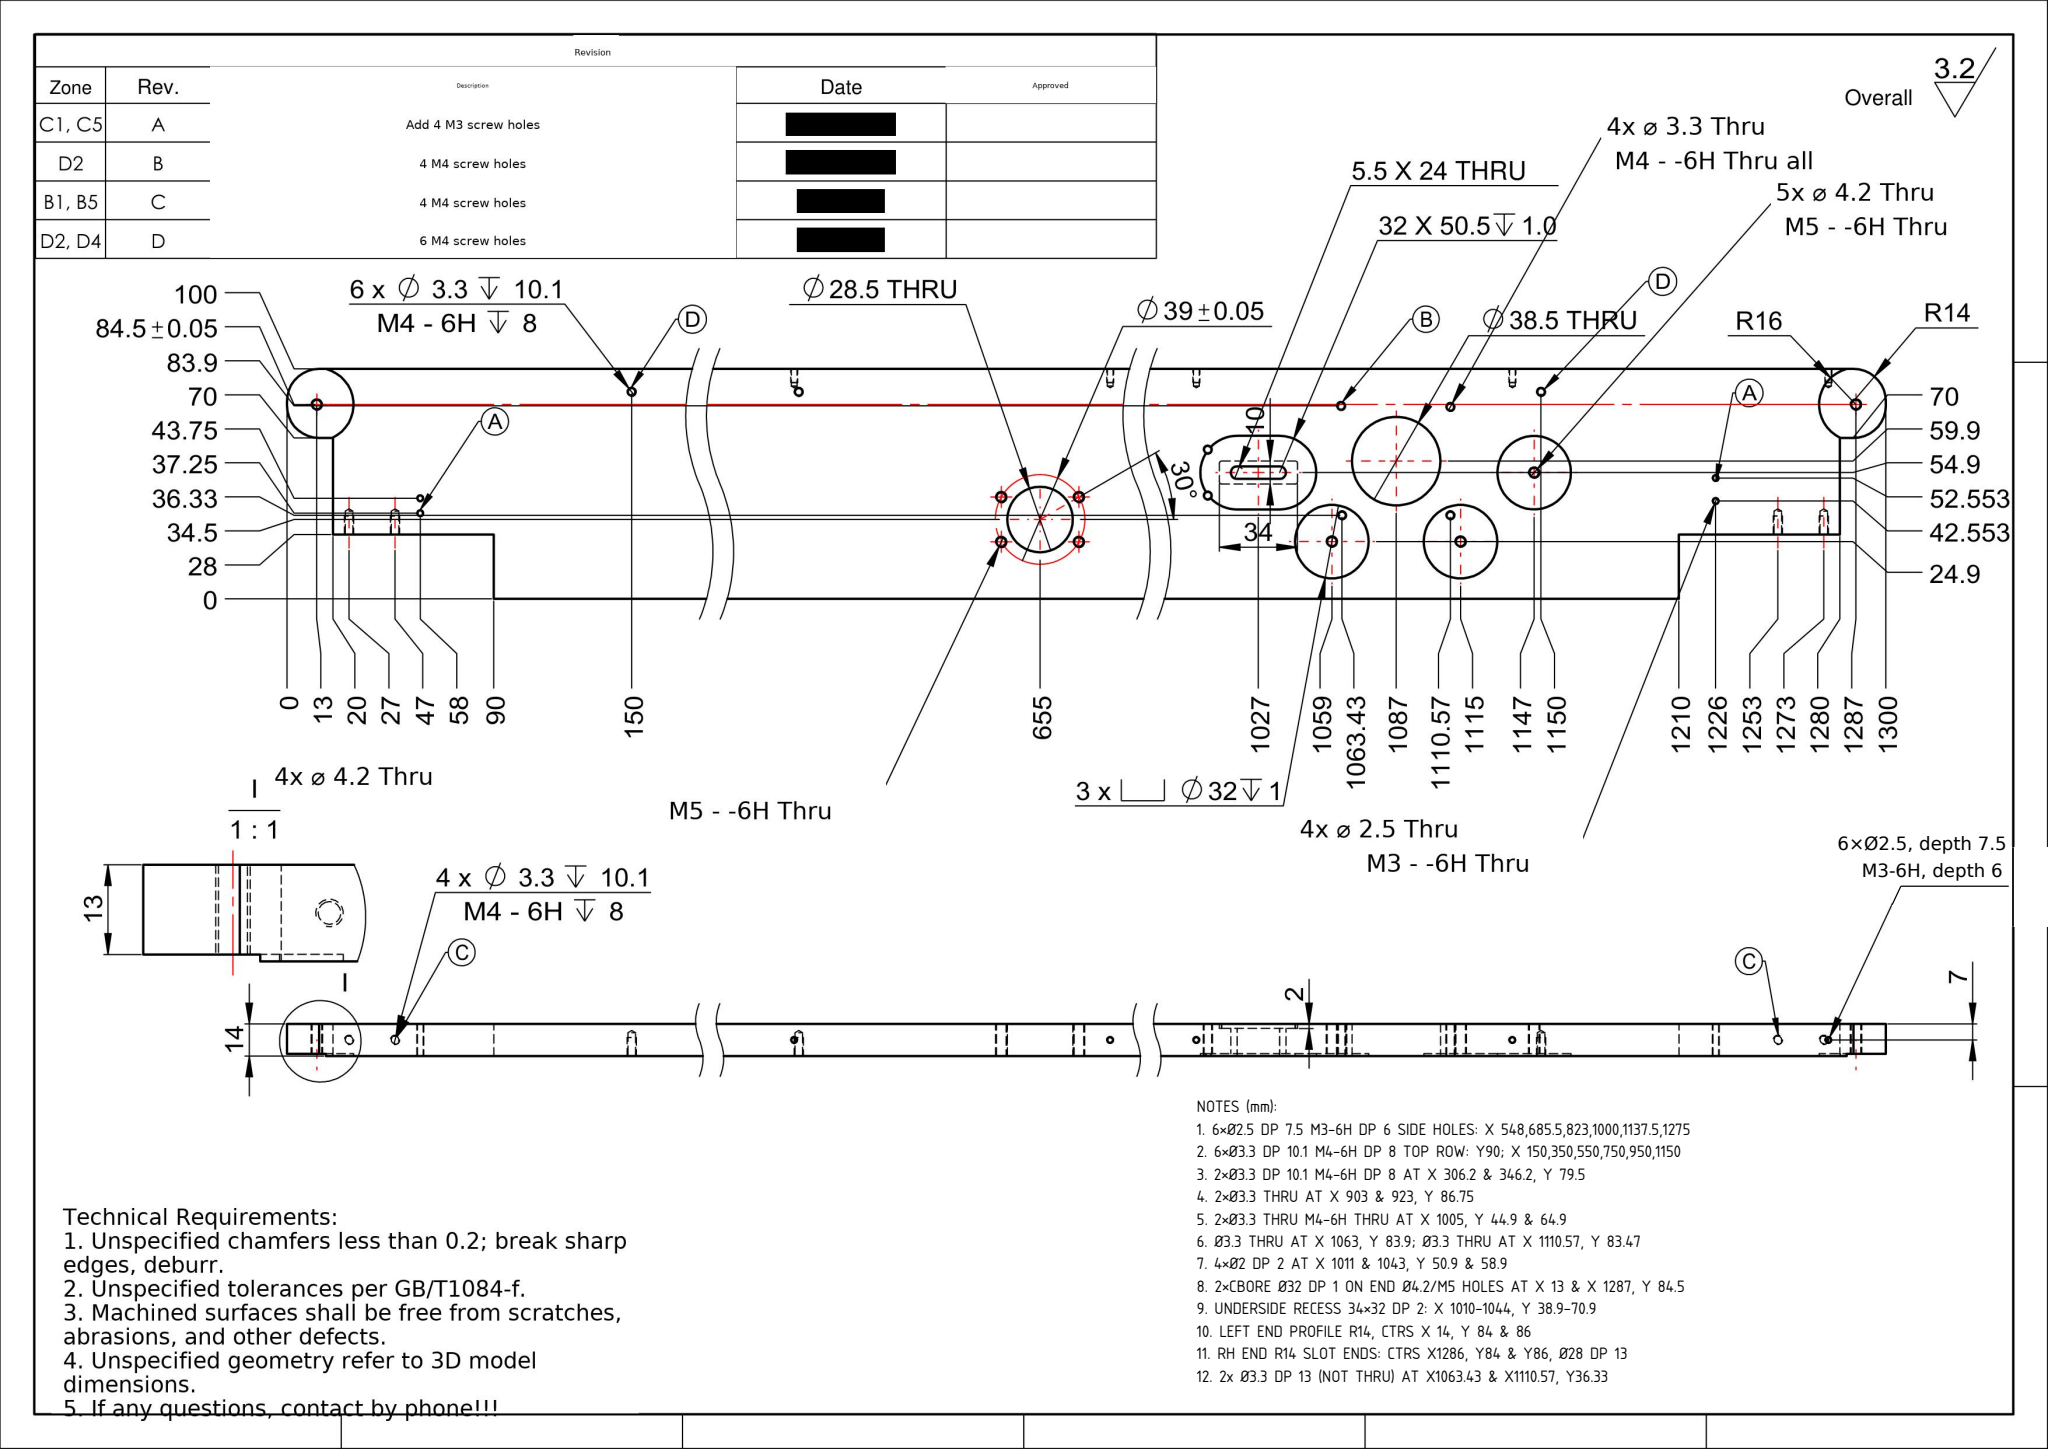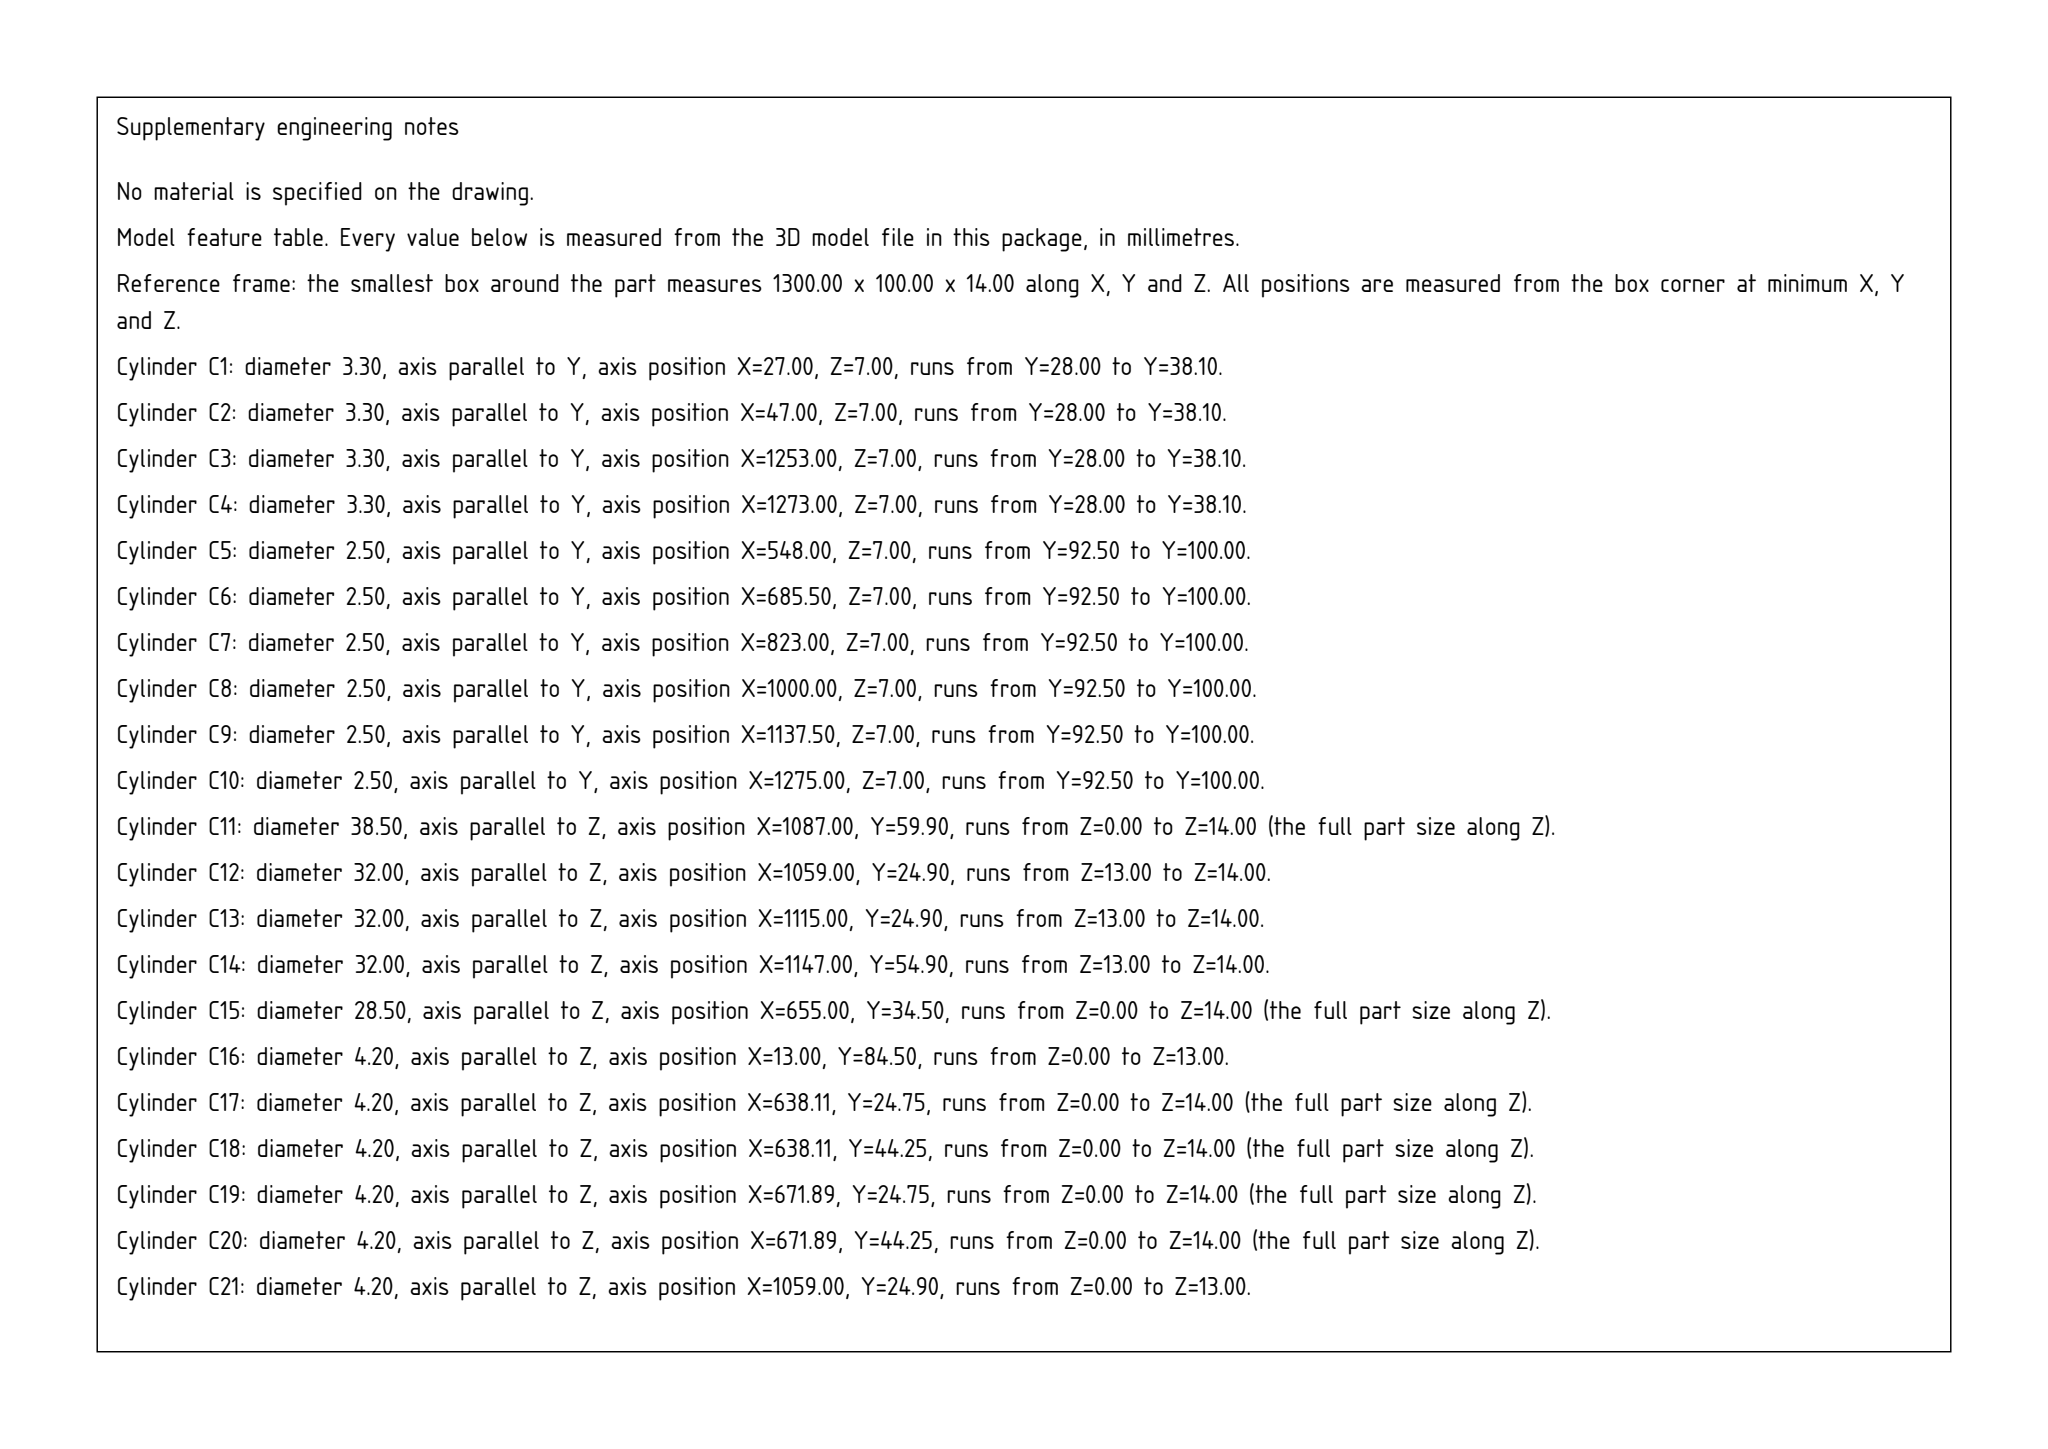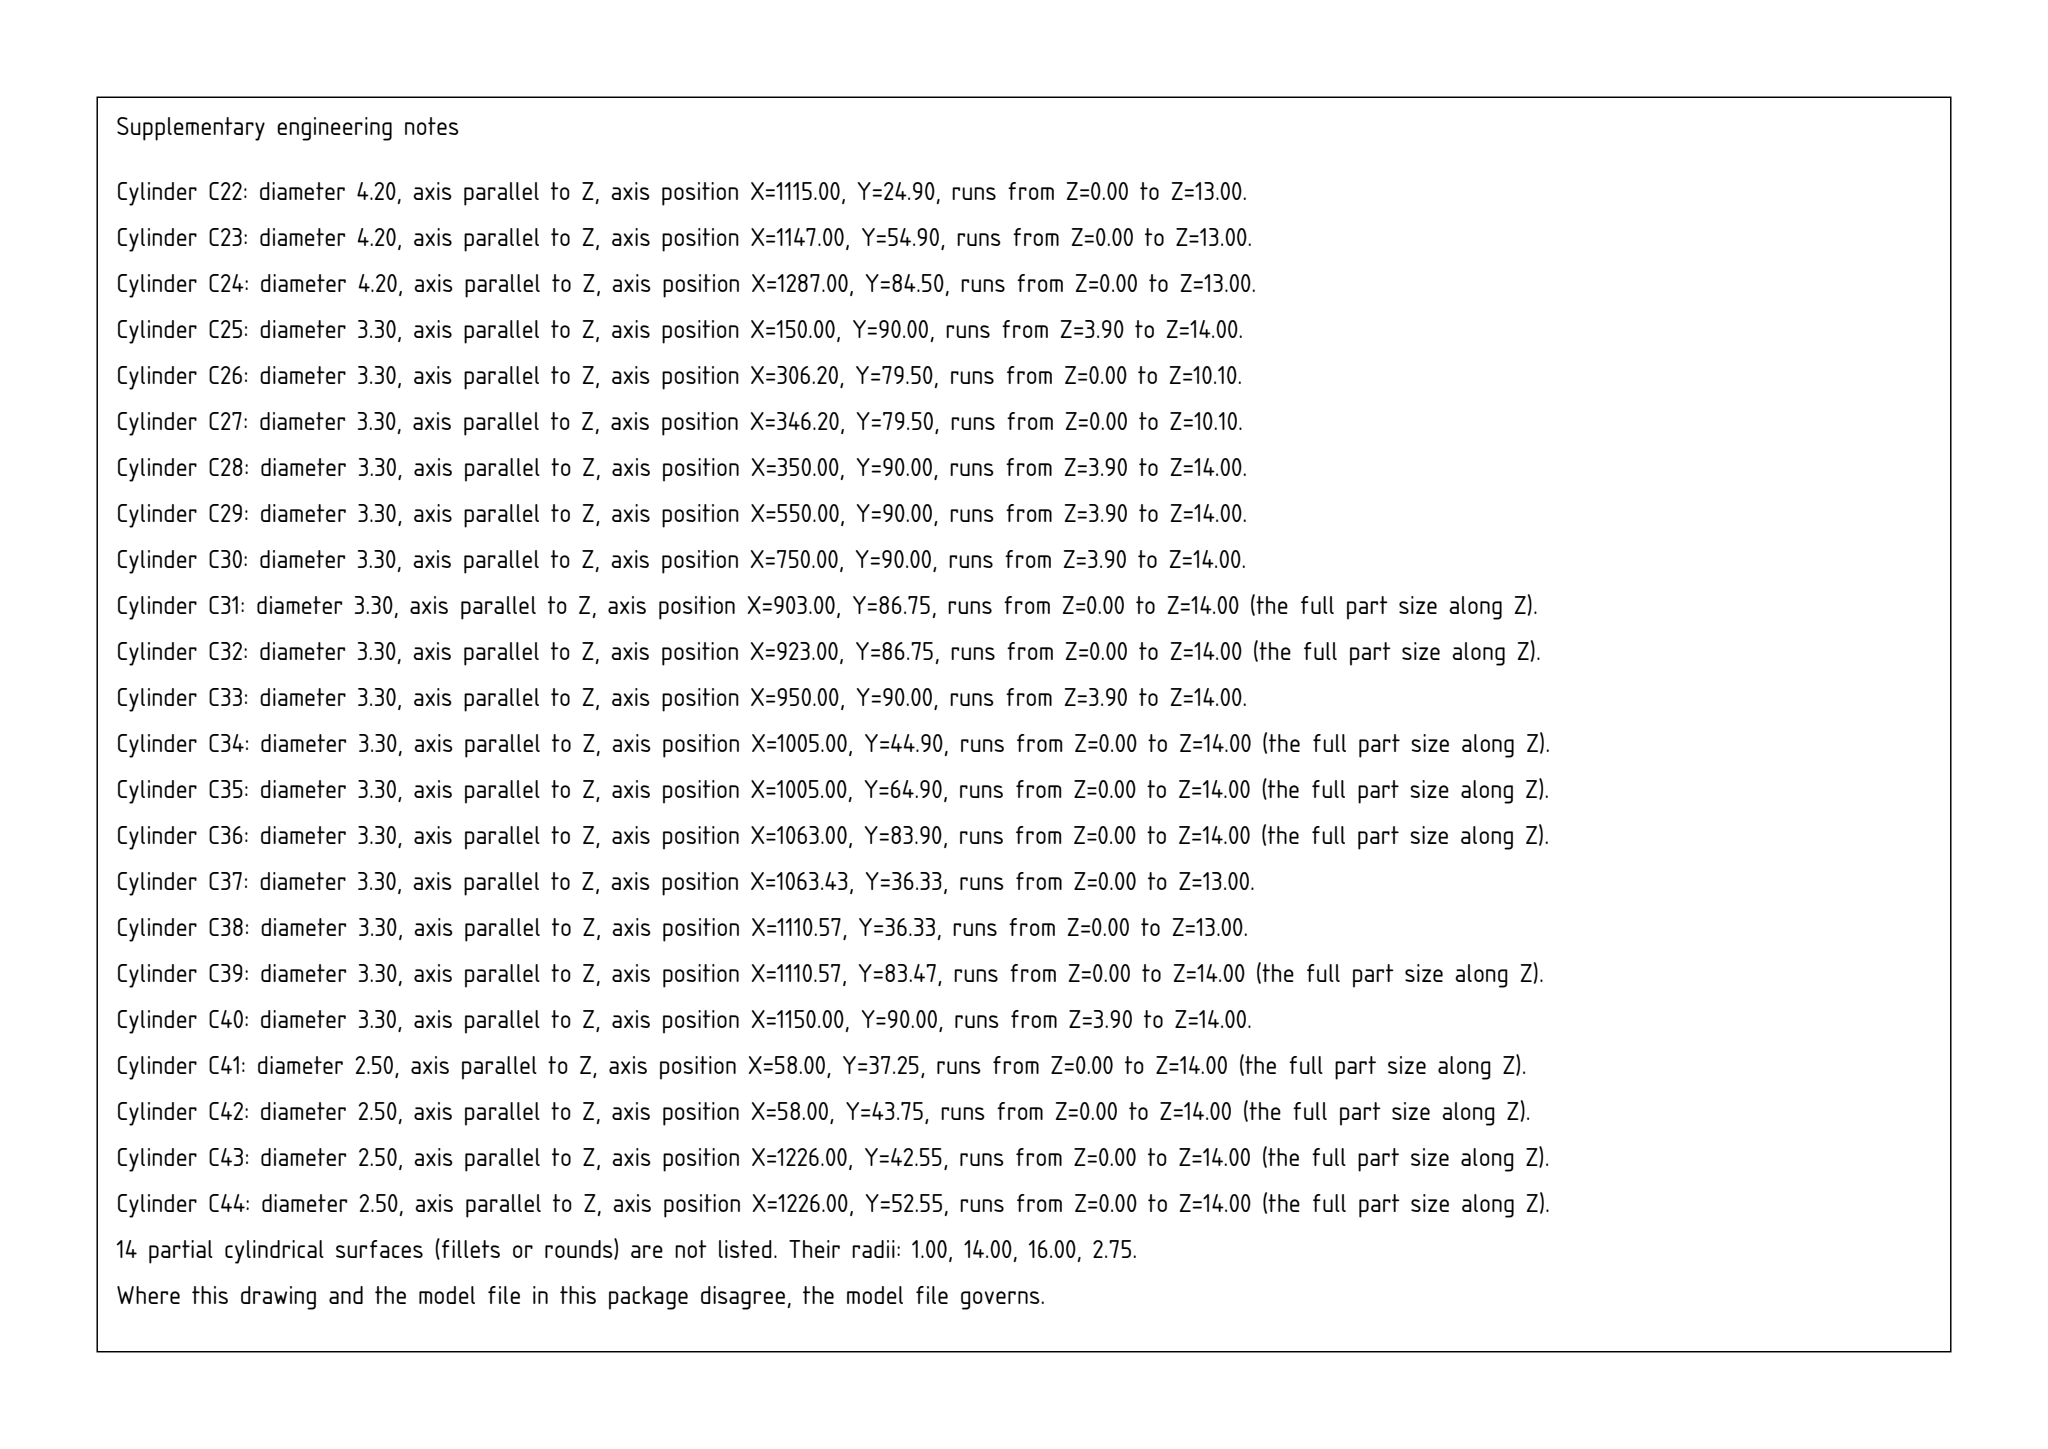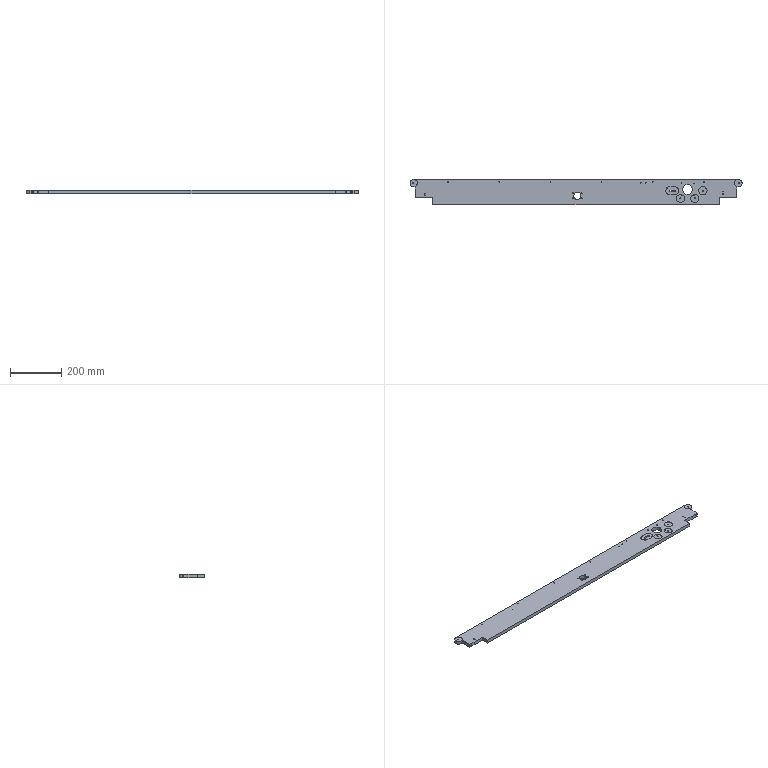Part | SolidWorks | mm | 1 solid | 172 faces | box 1300 x 100 x 14 mm | volume 1686884 mm3 | cylinder 107 | cone 36 | plane 29 | commonest cylinder face diameters 3.3 x40 2.5 x20 4.2 x18 32 x14 28 x4 2 x4 5.5 x3 28.5 x2
Drawing notes:
6×Ø2.5 DP 7.5 M3-6H DP 6 SIDE HOLES: X 548,685.5,823,1000,1137.5,1275 | from the solid: cyl dia2.5 axis y at x=548,685.5,823,1000,1137.5,1275, z=7, len 7.5
6×Ø3.3 DP 10.1 M4-6H DP 8 TOP ROW: Y90; X 150,350,550,750,950,1150 | from the solid: cyl dia3.3 axis z at (150/350/550/750/950/1150, 90), len 10.1
2×Ø3.3 DP 10.1 M4-6H DP 8 AT X 306.2 & 346.2, Y 79.5 | from the solid: cyl dia3.3 axis z at (306.2,79.5) and (346.2,79.5), len 10.1
2×Ø3.3 THRU AT X 903 & 923, Y 86.75 | from the solid: cyl dia3.3 axis z at (903,86.75),(923,86.75), len 14 = thru
2×Ø3.3 THRU M4-6H THRU AT X 1005, Y 44.9 & 64.9 | from the solid: cyl dia3.3 axis z at (1005,44.9),(1005,64.9), len 14 = thru
Ø3.3 THRU AT X 1063, Y 83.9; Ø3.3 THRU AT X 1110.57, Y 83.47 | from the solid: cyl dia3.3 axis z (1063,83.9) & (1110.57,83.47), len 14 = thru
4×Ø2 DP 2 AT X 1011 & 1043, Y 50.9 & 58.9 | from the solid: cyl dia2.0 axis z at (1011/1043, 50.9/58.9), len 2.0
2×CBORE Ø32 DP 1 ON END Ø4.2/M5 HOLES AT X 13 & X 1287, Y 84.5 | from the solid: cyl dia32 axis z at (13,84.5) and (1287,84.5), len 1.0
UNDERSIDE RECESS 34×32 DP 2: X 1010-1044, Y 38.9-70.9 | from the solid: x planes 1010 & 1044, y planes 38.9 & 70.9, z plane 2.0
LEFT END PROFILE R14, CTRS X 14, Y 84 & 86 | from the solid: cyl dia28 axis z at (14,84) and (14,86), len 13
RH END R14 SLOT ENDS: CTRS X1286, Y84 & Y86, Ø28 DP 13 | from the solid: cylinders [28.0,z,(1286.0,84.0),13.0] and [28.0,z,(1286.0,86.0),13.0]; mirrors LH pair at X14
2x Ø3.3 DP 13 (NOT THRU) AT X1063.43 & X1110.57, Y36.33 | from the solid: cylinders [3.3,z,(1063.43,36.33),13.0] and [3.3,z,(1110.57,36.33),13.0]; part thk 14 (z planes 0 & 14), 118° drill cone ref Ø3.3